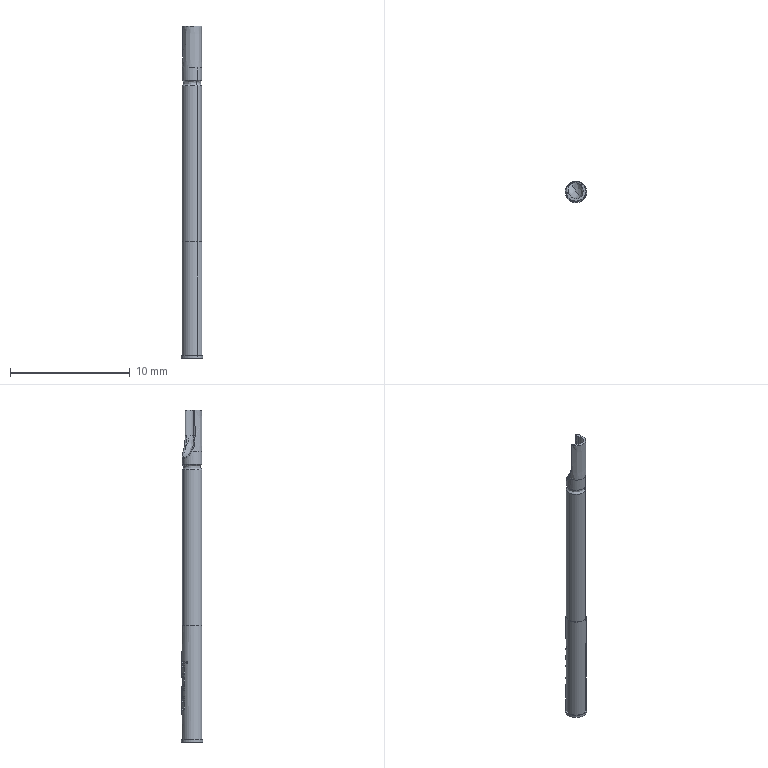Component | SolidWorks | 170423A4-GKS100-1_170423A4-KS-100_30_05-1 | 1 solid | 114 faces | box 1.8 x 1.8 x 27.7 mm | volume 20 mm3 | plane 47 | cylinder 35 | spline 29 | cone 3 | commonest cylinder face diameters 1.57 x15 1.67 x6 1.65 x4 0.2 x4 1.366 x2 1.8 x2 1.2 x2